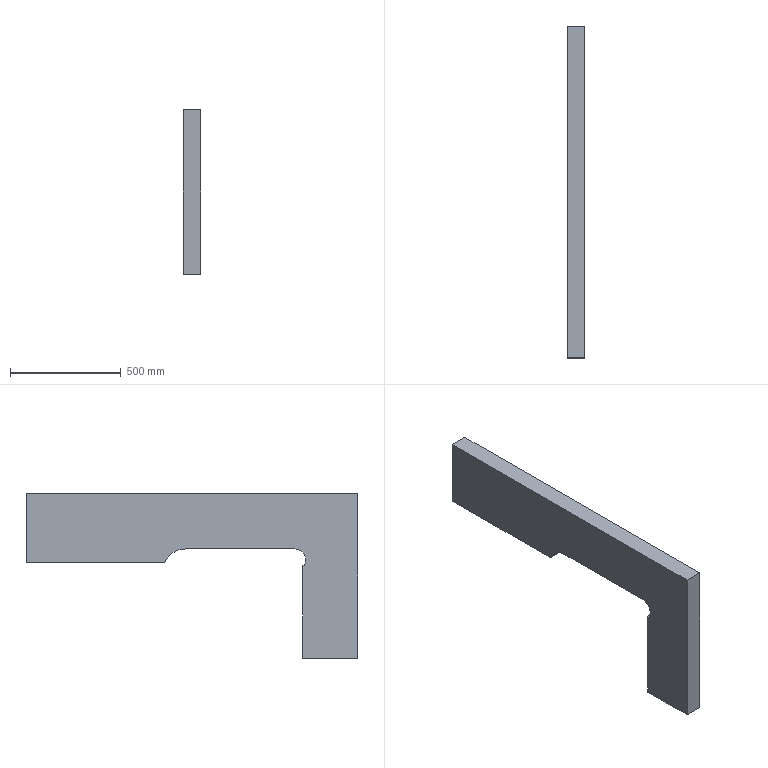Component | SolidWorks | JF21-80.1-1-3(_)-1-SOLID17-1 | 1 solid | 12 faces | box 80 x 1499 x 745 mm | volume 43121801 mm3 | plane 10 | cylinder 2 | commonest cylinder face diameters 200 x1 100 x1
STEP:
#1=CARTESIAN_POINT('',(15.748,-62.205,-7.677));
#2=VERTEX_POINT('',#1);
#3=CARTESIAN_POINT('',(15.748,-72.047,-7.677));
#4=VERTEX_POINT('',#3);
#5=CARTESIAN_POINT('',(15.748,-72.047,-7.677));
#6=DIRECTION('',(0.,-1.,0.));
#7=VECTOR('',#6,39.37);
#8=LINE('',#5,#7);
#9=EDGE_CURVE('',#2,#4,#8,.T.);
#10=ORIENTED_EDGE('',*,*,#9,.T.);
#11=CARTESIAN_POINT('',(12.598,-72.047,-7.677));
#12=VERTEX_POINT('',#11);
#13=CARTESIAN_POINT('',(12.598,-72.047,-7.677));
#14=DIRECTION('',(1.,0.,0.));
#15=VECTOR('',#14,39.37);
#16=LINE('',#13,#15);
#17=EDGE_CURVE('',#12,#4,#16,.T.);
#18=ORIENTED_EDGE('',*,*,#17,.F.);
#19=CARTESIAN_POINT('',(12.598,-62.205,-7.677));
#20=VERTEX_POINT('',#19);
#21=CARTESIAN_POINT('',(12.598,-72.047,-7.677));
#22=DIRECTION('',(0.,-1.,0.));
#23=VECTOR('',#22,39.37);
#24=LINE('',#21,#23);
#25=EDGE_CURVE('',#20,#12,#24,.T.);
#26=ORIENTED_EDGE('',*,*,#25,.F.);
#27=CARTESIAN_POINT('',(12.598,-62.205,-7.677));
#28=DIRECTION('',(1.,0.,0.));
#29=VECTOR('',#28,39.37);
#30=LINE('',#27,#29);
#31=EDGE_CURVE('',#20,#2,#30,.T.);
#32=ORIENTED_EDGE('',*,*,#31,.T.);
#33=EDGE_LOOP('',(#10,#18,#26,#32));
#34=FACE_OUTER_BOUND('',#33,.T.);
#35=CARTESIAN_POINT('',(12.598,-72.047,-7.677));
#36=DIRECTION('',(0.,0.,1.));
#37=DIRECTION('',(-1.,0.,0.));
#38=AXIS2_PLACEMENT_3D('',#35,#36,#37);
#39=PLANE('',#38);
#40=ADVANCED_FACE('',(#34),#39,.F.);
#41=CARTESIAN_POINT('',(15.748,-72.047,21.654));
#42=VERTEX_POINT('',#41);
#43=CARTESIAN_POINT('',(15.748,-72.047,-7.677));
#44=DIRECTION('',(0.,0.,1.));
#45=VECTOR('',#44,39.37);
#46=LINE('',#43,#45);
#47=EDGE_CURVE('',#4,#42,#46,.T.);
#48=ORIENTED_EDGE('',*,*,#47,.T.);
#49=CARTESIAN_POINT('',(12.598,-72.047,21.654));
#50=VERTEX_POINT('',#49);
#51=CARTESIAN_POINT('',(12.598,-72.047,21.654));
#52=DIRECTION('',(1.,0.,0.));
#53=VECTOR('',#52,39.37);
#54=LINE('',#51,#53);
#55=EDGE_CURVE('',#50,#42,#54,.T.);
#56=ORIENTED_EDGE('',*,*,#55,.F.);
#57=CARTESIAN_POINT('',(12.598,-72.047,-7.677));
#58=DIRECTION('',(0.,0.,1.));
#59=VECTOR('',#58,39.37);
#60=LINE('',#57,#59);
#61=EDGE_CURVE('',#12,#50,#60,.T.);
#62=ORIENTED_EDGE('',*,*,#61,.F.);
#63=ORIENTED_EDGE('',*,*,#17,.T.);
#64=EDGE_LOOP('',(#48,#56,#62,#63));
#65=FACE_OUTER_BOUND('',#64,.T.);
#66=CARTESIAN_POINT('',(12.598,-72.047,-7.677));
#67=DIRECTION('',(0.,1.,0.));
#68=DIRECTION('',(0.,0.,-1.));
#69=AXIS2_PLACEMENT_3D('',#66,#67,#68);
#70=PLANE('',#69);
#71=ADVANCED_FACE('',(#65),#70,.F.);
#72=CARTESIAN_POINT('',(15.748,-13.031,21.654));
#73=VERTEX_POINT('',#72);
#74=CARTESIAN_POINT('',(15.748,-72.047,21.654));
#75=DIRECTION('',(0.,1.,0.));
#76=VECTOR('',#75,39.37);
#77=LINE('',#74,#76);
#78=EDGE_CURVE('',#42,#73,#77,.T.);
#79=ORIENTED_EDGE('',*,*,#78,.T.);
#80=CARTESIAN_POINT('',(12.598,-13.031,21.654));
#81=VERTEX_POINT('',#80);
#82=CARTESIAN_POINT('',(12.598,-13.031,21.654));
#83=DIRECTION('',(1.,0.,0.));
#84=VECTOR('',#83,39.37);
#85=LINE('',#82,#84);
#86=EDGE_CURVE('',#81,#73,#85,.T.);
#87=ORIENTED_EDGE('',*,*,#86,.F.);
#88=CARTESIAN_POINT('',(12.598,-72.047,21.654));
#89=DIRECTION('',(0.,1.,0.));
#90=VECTOR('',#89,39.37);
#91=LINE('',#88,#90);
#92=EDGE_CURVE('',#50,#81,#91,.T.);
#93=ORIENTED_EDGE('',*,*,#92,.F.);
#94=ORIENTED_EDGE('',*,*,#55,.T.);
#95=EDGE_LOOP('',(#79,#87,#93,#94));
#96=FACE_OUTER_BOUND('',#95,.T.);
#97=CARTESIAN_POINT('',(12.598,-72.047,21.654));
#98=DIRECTION('',(0.,0.,-1.));
#99=DIRECTION('',(0.,-1.,-0.));
#100=AXIS2_PLACEMENT_3D('',#97,#98,#99);
#101=PLANE('',#100);
#102=ADVANCED_FACE('',(#96),#101,.F.);
#103=CARTESIAN_POINT('',(15.748,-13.031,9.331));
#104=VERTEX_POINT('',#103);
#105=CARTESIAN_POINT('',(15.748,-13.031,21.654));
#106=DIRECTION('',(0.,-0.,-1.));
#107=VECTOR('',#106,39.37);
#108=LINE('',#105,#107);
#109=EDGE_CURVE('',#73,#104,#108,.T.);
#110=ORIENTED_EDGE('',*,*,#109,.T.);
#111=CARTESIAN_POINT('',(12.598,-13.031,9.331));
#112=VERTEX_POINT('',#111);
#113=CARTESIAN_POINT('',(12.598,-13.031,9.331));
#114=DIRECTION('',(1.,0.,0.));
#115=VECTOR('',#114,39.37);
#116=LINE('',#113,#115);
#117=EDGE_CURVE('',#112,#104,#116,.T.);
#118=ORIENTED_EDGE('',*,*,#117,.F.);
#119=CARTESIAN_POINT('',(12.598,-13.031,21.654));
#120=DIRECTION('',(0.,-0.,-1.));
#121=VECTOR('',#120,39.37);
#122=LINE('',#119,#121);
#123=EDGE_CURVE('',#81,#112,#122,.T.);
#124=ORIENTED_EDGE('',*,*,#123,.F.);
#125=ORIENTED_EDGE('',*,*,#86,.T.);
#126=EDGE_LOOP('',(#110,#118,#124,#125));
#127=FACE_OUTER_BOUND('',#126,.T.);
#128=CARTESIAN_POINT('',(12.598,-13.031,21.654));
#129=DIRECTION('',(0.,-1.,0.));
#130=DIRECTION('',(0.,0.,1.));
#131=AXIS2_PLACEMENT_3D('',#128,#129,#130);
#132=PLANE('',#131);
#133=ADVANCED_FACE('',(#127),#132,.F.);
#134=CARTESIAN_POINT('',(15.748,-37.681,9.331));
#135=VERTEX_POINT('',#134);
#136=CARTESIAN_POINT('',(15.748,-13.031,9.331));
#137=DIRECTION('',(0.,-1.,0.));
#138=VECTOR('',#137,39.37);
#139=LINE('',#136,#138);
#140=EDGE_CURVE('',#104,#135,#139,.T.);
#141=ORIENTED_EDGE('',*,*,#140,.T.);
#142=CARTESIAN_POINT('',(12.598,-37.681,9.331));
#143=VERTEX_POINT('',#142);
#144=CARTESIAN_POINT('',(12.598,-37.681,9.331));
#145=DIRECTION('',(1.,0.,0.));
#146=VECTOR('',#145,39.37);
#147=LINE('',#144,#146);
#148=EDGE_CURVE('',#143,#135,#147,.T.);
#149=ORIENTED_EDGE('',*,*,#148,.F.);
#150=CARTESIAN_POINT('',(12.598,-13.031,9.331));
#151=DIRECTION('',(0.,-1.,0.));
#152=VECTOR('',#151,39.37);
#153=LINE('',#150,#152);
#154=EDGE_CURVE('',#112,#143,#153,.T.);
#155=ORIENTED_EDGE('',*,*,#154,.F.);
#156=ORIENTED_EDGE('',*,*,#117,.T.);
#157=EDGE_LOOP('',(#141,#149,#155,#156));
#158=FACE_OUTER_BOUND('',#157,.T.);
#159=CARTESIAN_POINT('',(12.598,-13.031,9.331));
#160=DIRECTION('',(0.,0.,1.));
#161=DIRECTION('',(0.,1.,-0.));
#162=AXIS2_PLACEMENT_3D('',#159,#160,#161);
#163=PLANE('',#162);
#164=ADVANCED_FACE('',(#158),#163,.F.);
#165=CARTESIAN_POINT('',(15.748,-41.339,11.811));
#166=VERTEX_POINT('',#165);
#167=CARTESIAN_POINT('',(15.748,-41.339,7.874));
#168=DIRECTION('',(1.,0.,0.));
#169=DIRECTION('',(0.,0.,1.));
#170=AXIS2_PLACEMENT_3D('',#167,#168,#169);
#171=CIRCLE('',#170,3.937);
#172=EDGE_CURVE('',#135,#166,#171,.T.);
#173=ORIENTED_EDGE('',*,*,#172,.T.);
#174=CARTESIAN_POINT('',(12.598,-41.339,11.811));
#175=VERTEX_POINT('',#174);
#176=CARTESIAN_POINT('',(12.598,-41.339,11.811));
#177=DIRECTION('',(1.,0.,0.));
#178=VECTOR('',#177,39.37);
#179=LINE('',#176,#178);
#180=EDGE_CURVE('',#175,#166,#179,.T.);
#181=ORIENTED_EDGE('',*,*,#180,.F.);
#182=CARTESIAN_POINT('',(12.598,-41.339,7.874));
#183=DIRECTION('',(1.,0.,0.));
#184=DIRECTION('',(0.,0.,1.));
#185=AXIS2_PLACEMENT_3D('',#182,#183,#184);
#186=CIRCLE('',#185,3.937);
#187=EDGE_CURVE('',#143,#175,#186,.T.);
#188=ORIENTED_EDGE('',*,*,#187,.F.);
#189=ORIENTED_EDGE('',*,*,#148,.T.);
#190=EDGE_LOOP('',(#173,#181,#188,#189));
#191=FACE_OUTER_BOUND('',#190,.T.);
#192=CARTESIAN_POINT('',(12.598,-41.339,7.874));
#193=DIRECTION('',(1.,0.,0.));
#194=DIRECTION('',(0.,0.,1.));
#195=AXIS2_PLACEMENT_3D('',#192,#193,#194);
#196=CYLINDRICAL_SURFACE('',#195,3.937);
#197=ADVANCED_FACE('',(#191),#196,.F.);
#198=CARTESIAN_POINT('',(15.748,-60.827,11.811));
#199=VERTEX_POINT('',#198);
#200=CARTESIAN_POINT('',(15.748,-60.827,11.811));
#201=DIRECTION('',(0.,-1.,-0.));
#202=VECTOR('',#201,39.37);
#203=LINE('',#200,#202);
#204=EDGE_CURVE('',#166,#199,#203,.T.);
#205=ORIENTED_EDGE('',*,*,#204,.T.);
#206=CARTESIAN_POINT('',(12.598,-60.827,11.811));
#207=VERTEX_POINT('',#206);
#208=CARTESIAN_POINT('',(12.598,-60.827,11.811));
#209=DIRECTION('',(1.,0.,0.));
#210=VECTOR('',#209,39.37);
#211=LINE('',#208,#210);
#212=EDGE_CURVE('',#207,#199,#211,.T.);
#213=ORIENTED_EDGE('',*,*,#212,.F.);
#214=CARTESIAN_POINT('',(12.598,-60.827,11.811));
#215=DIRECTION('',(0.,-1.,-0.));
#216=VECTOR('',#215,39.37);
#217=LINE('',#214,#216);
#218=EDGE_CURVE('',#175,#207,#217,.T.);
#219=ORIENTED_EDGE('',*,*,#218,.F.);
#220=ORIENTED_EDGE('',*,*,#180,.T.);
#221=EDGE_LOOP('',(#205,#213,#219,#220));
#222=FACE_OUTER_BOUND('',#221,.T.);
#223=CARTESIAN_POINT('',(12.598,-60.827,11.811));
#224=DIRECTION('',(0.,-0.,1.));
#225=DIRECTION('',(0.,1.,0.));
#226=AXIS2_PLACEMENT_3D('',#223,#224,#225);
#227=PLANE('',#226);
#228=ADVANCED_FACE('',(#222),#227,.F.);
#229=CARTESIAN_POINT('',(15.748,-62.532,8.858));
#230=VERTEX_POINT('',#229);
#231=CARTESIAN_POINT('',(15.748,-60.827,9.843));
#232=DIRECTION('',(1.,0.,0.));
#233=DIRECTION('',(0.,0.,1.));
#234=AXIS2_PLACEMENT_3D('',#231,#232,#233);
#235=CIRCLE('',#234,1.969);
#236=EDGE_CURVE('',#199,#230,#235,.T.);
#237=ORIENTED_EDGE('',*,*,#236,.T.);
#238=CARTESIAN_POINT('',(12.598,-62.532,8.858));
#239=VERTEX_POINT('',#238);
#240=CARTESIAN_POINT('',(12.598,-62.532,8.858));
#241=DIRECTION('',(1.,0.,0.));
#242=VECTOR('',#241,39.37);
#243=LINE('',#240,#242);
#244=EDGE_CURVE('',#239,#230,#243,.T.);
#245=ORIENTED_EDGE('',*,*,#244,.F.);
#246=CARTESIAN_POINT('',(12.598,-60.827,9.843));
#247=DIRECTION('',(1.,0.,0.));
#248=DIRECTION('',(0.,0.,1.));
#249=AXIS2_PLACEMENT_3D('',#246,#247,#248);
#250=CIRCLE('',#249,1.969);
#251=EDGE_CURVE('',#207,#239,#250,.T.);
#252=ORIENTED_EDGE('',*,*,#251,.F.);
#253=ORIENTED_EDGE('',*,*,#212,.T.);
#254=EDGE_LOOP('',(#237,#245,#252,#253));
#255=FACE_OUTER_BOUND('',#254,.T.);
#256=CARTESIAN_POINT('',(12.598,-60.827,9.843));
#257=DIRECTION('',(1.,0.,0.));
#258=DIRECTION('',(0.,0.,1.));
#259=AXIS2_PLACEMENT_3D('',#256,#257,#258);
#260=CYLINDRICAL_SURFACE('',#259,1.969);
#261=ADVANCED_FACE('',(#255),#260,.F.);
#262=CARTESIAN_POINT('',(15.748,-62.205,8.858));
#263=VERTEX_POINT('',#262);
#264=CARTESIAN_POINT('',(15.748,-62.205,8.858));
#265=DIRECTION('',(0.,1.,0.));
#266=VECTOR('',#265,39.37);
#267=LINE('',#264,#266);
#268=EDGE_CURVE('',#230,#263,#267,.T.);
#269=ORIENTED_EDGE('',*,*,#268,.T.);
#270=CARTESIAN_POINT('',(12.598,-62.205,8.858));
#271=VERTEX_POINT('',#270);
#272=CARTESIAN_POINT('',(12.598,-62.205,8.858));
#273=DIRECTION('',(1.,0.,0.));
#274=VECTOR('',#273,39.37);
#275=LINE('',#272,#274);
#276=EDGE_CURVE('',#271,#263,#275,.T.);
#277=ORIENTED_EDGE('',*,*,#276,.F.);
#278=CARTESIAN_POINT('',(12.598,-62.205,8.858));
#279=DIRECTION('',(0.,1.,0.));
#280=VECTOR('',#279,39.37);
#281=LINE('',#278,#280);
#282=EDGE_CURVE('',#239,#271,#281,.T.);
#283=ORIENTED_EDGE('',*,*,#282,.F.);
#284=ORIENTED_EDGE('',*,*,#244,.T.);
#285=EDGE_LOOP('',(#269,#277,#283,#284));
#286=FACE_OUTER_BOUND('',#285,.T.);
#287=CARTESIAN_POINT('',(12.598,-62.205,8.858));
#288=DIRECTION('',(0.,0.,-1.));
#289=DIRECTION('',(1.,0.,0.));
#290=AXIS2_PLACEMENT_3D('',#287,#288,#289);
#291=PLANE('',#290);
#292=ADVANCED_FACE('',(#286),#291,.F.);
#293=CARTESIAN_POINT('',(15.748,-62.205,-7.677));
#294=DIRECTION('',(0.,0.,-1.));
#295=VECTOR('',#294,39.37);
#296=LINE('',#293,#295);
#297=EDGE_CURVE('',#263,#2,#296,.T.);
#298=ORIENTED_EDGE('',*,*,#297,.T.);
#299=ORIENTED_EDGE('',*,*,#31,.F.);
#300=CARTESIAN_POINT('',(12.598,-62.205,-7.677));
#301=DIRECTION('',(0.,0.,-1.));
#302=VECTOR('',#301,39.37);
#303=LINE('',#300,#302);
#304=EDGE_CURVE('',#271,#20,#303,.T.);
#305=ORIENTED_EDGE('',*,*,#304,.F.);
#306=ORIENTED_EDGE('',*,*,#276,.T.);
#307=EDGE_LOOP('',(#298,#299,#305,#306));
#308=FACE_OUTER_BOUND('',#307,.T.);
#309=CARTESIAN_POINT('',(12.598,-62.205,-7.677));
#310=DIRECTION('',(0.,-1.,0.));
#311=DIRECTION('',(0.,0.,1.));
#312=AXIS2_PLACEMENT_3D('',#309,#310,#311);
#313=PLANE('',#312);
#314=ADVANCED_FACE('',(#308),#313,.F.);
#315=ORIENTED_EDGE('',*,*,#25,.T.);
#316=ORIENTED_EDGE('',*,*,#61,.T.);
#317=ORIENTED_EDGE('',*,*,#92,.T.);
#318=ORIENTED_EDGE('',*,*,#123,.T.);
#319=ORIENTED_EDGE('',*,*,#154,.T.);
#320=ORIENTED_EDGE('',*,*,#187,.T.);
#321=ORIENTED_EDGE('',*,*,#218,.T.);
#322=ORIENTED_EDGE('',*,*,#251,.T.);
#323=ORIENTED_EDGE('',*,*,#282,.T.);
#324=ORIENTED_EDGE('',*,*,#304,.T.);
#325=EDGE_LOOP('',(#315,#316,#317,#318,#319,#320,#321,#322,#323,#324));
#326=FACE_OUTER_BOUND('',#325,.T.);
#327=CARTESIAN_POINT('',(12.598,-60.827,9.843));
#328=DIRECTION('',(-1.,0.,0.));
#329=DIRECTION('',(0.,0.,-1.));
#330=AXIS2_PLACEMENT_3D('',#327,#328,#329);
#331=PLANE('',#330);
#332=ADVANCED_FACE('',(#326),#331,.T.);
#333=ORIENTED_EDGE('',*,*,#9,.F.);
#334=ORIENTED_EDGE('',*,*,#297,.F.);
#335=ORIENTED_EDGE('',*,*,#268,.F.);
#336=ORIENTED_EDGE('',*,*,#236,.F.);
#337=ORIENTED_EDGE('',*,*,#204,.F.);
#338=ORIENTED_EDGE('',*,*,#172,.F.);
#339=ORIENTED_EDGE('',*,*,#140,.F.);
#340=ORIENTED_EDGE('',*,*,#109,.F.);
#341=ORIENTED_EDGE('',*,*,#78,.F.);
#342=ORIENTED_EDGE('',*,*,#47,.F.);
#343=EDGE_LOOP('',(#333,#334,#335,#336,#337,#338,#339,#340,#341,#342));
#344=FACE_OUTER_BOUND('',#343,.T.);
#345=CARTESIAN_POINT('',(15.748,-60.827,9.843));
#346=DIRECTION('',(-1.,0.,0.));
#347=DIRECTION('',(0.,0.,-1.));
#348=AXIS2_PLACEMENT_3D('',#345,#346,#347);
#349=PLANE('',#348);
#350=ADVANCED_FACE('',(#344),#349,.F.);
#351=CLOSED_SHELL('',(#40,#71,#102,#133,#164,#197,#228,#261,#292,#314,#332,#350));
#352=MANIFOLD_SOLID_BREP('',#351);
#353=CARTESIAN_POINT('',(0.,0.,0.));
#354=DIRECTION('',(0.,0.,1.));
#355=DIRECTION('',(1.,0.,0.));
#356=AXIS2_PLACEMENT_3D('',#353,#354,#355);
#357=(LENGTH_UNIT()NAMED_UNIT(*)SI_UNIT($,.METRE.));
#358=LENGTH_MEASURE_WITH_UNIT(LENGTH_MEASURE(0.0254),#357);
#359=DIMENSIONAL_EXPONENTS(1.,0.,0.,0.,0.,0.,0.);
#360=(CONVERSION_BASED_UNIT('',#358)LENGTH_UNIT()NAMED_UNIT(#359));
#361=UNCERTAINTY_MEASURE_WITH_UNIT(LENGTH_MEASURE(0.00001),#360,'','');
#362=(NAMED_UNIT(*)PLANE_ANGLE_UNIT()SI_UNIT($,.RADIAN.));
#363=(NAMED_UNIT(*)SI_UNIT($,.STERADIAN.)SOLID_ANGLE_UNIT());
#364=(GEOMETRIC_REPRESENTATION_CONTEXT(3)GLOBAL_UNCERTAINTY_ASSIGNED_CONTEXT((#361))GLOBAL_UNIT_ASSIGNED_CONTEXT((#360,#362,#363))REPRESENTATION_CONTEXT('',''));
#365=ADVANCED_BREP_SHAPE_REPRESENTATION('',(#352,#356),#364);
#366=COLOUR_RGB('',0.7922,0.8196,0.9333);
#367=FILL_AREA_STYLE_COLOUR('',#366);
#368=FILL_AREA_STYLE('',(#367));
#369=SURFACE_STYLE_FILL_AREA(#368);
#370=SURFACE_SIDE_STYLE('',(#369));
#371=SURFACE_STYLE_USAGE(.BOTH.,#370);
#372=PRESENTATION_STYLE_ASSIGNMENT((#371));
#373=STYLED_ITEM('',(#372),#352);
#374=PRESENTATION_LAYER_ASSIGNMENT('','',(#373));
#375=(LENGTH_UNIT()NAMED_UNIT(*)SI_UNIT($,.METRE.));
#376=LENGTH_MEASURE_WITH_UNIT(LENGTH_MEASURE(0.0254),#375);
#377=DIMENSIONAL_EXPONENTS(1.,0.,0.,0.,0.,0.,0.);
#378=(CONVERSION_BASED_UNIT('',#376)LENGTH_UNIT()NAMED_UNIT(#377));
#379=UNCERTAINTY_MEASURE_WITH_UNIT(LENGTH_MEASURE(0.00001),#378,'','');
#380=(NAMED_UNIT(*)PLANE_ANGLE_UNIT()SI_UNIT($,.RADIAN.));
#381=(NAMED_UNIT(*)SI_UNIT($,.STERADIAN.)SOLID_ANGLE_UNIT());
#382=(GEOMETRIC_REPRESENTATION_CONTEXT(3)GLOBAL_UNCERTAINTY_ASSIGNED_CONTEXT((#379))GLOBAL_UNIT_ASSIGNED_CONTEXT((#378,#380,#381))REPRESENTATION_CONTEXT('',''));
#383=MECHANICAL_DESIGN_GEOMETRIC_PRESENTATION_REPRESENTATION('',(#373),#382);